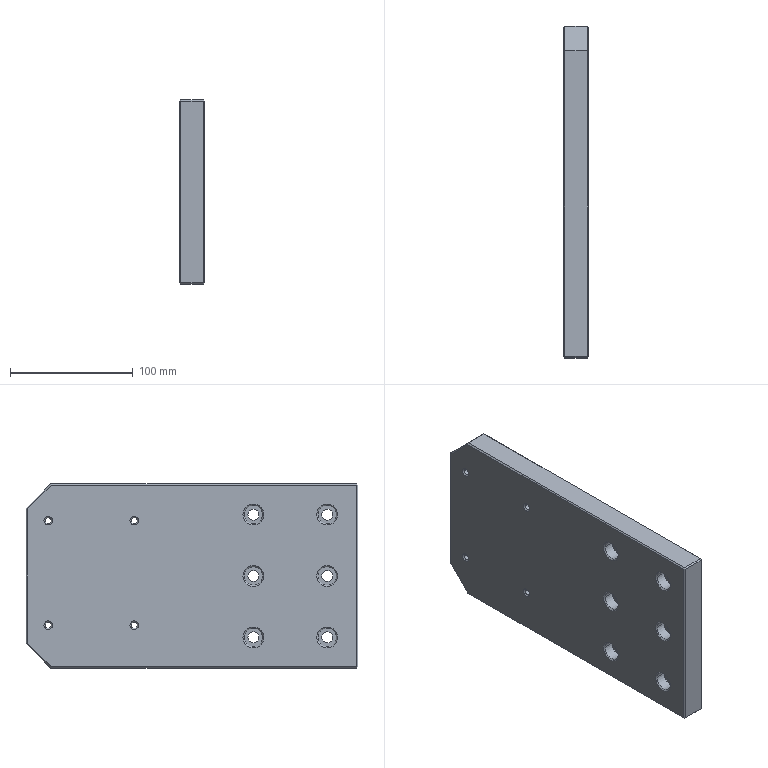Component | SolidWorks | CutterFixingPlateA-1 | 1 solid | 104 faces | box 20 x 270 x 150 mm | volume 785545 mm3 | cone 40 | cylinder 32 | plane 32 | commonest cylinder face diameters 15 x12 9 x12 5 x8 | material 1060 Alloy
build123d program:
from build123d import *

# Parameters (mm, degrees)
BOSS_EXTRUDE1_DEPTH                                = 20
M6_TAPPED_HOLE1_D                                  = 5
CHAMFER1_SIZE                                      = 20
SKETCH6_W                                          = 478.656
SKETCH6_H                                          = 357.372
CUT_EXTRUDE1_DEPTH                                 = 463.52
HOLE_SIZE_ACCORDING_TO_TYPE_OF_HEXAGON_D           = 9
HOLE_SIZE_ACCORDING_TO_TYPE_OF_HEXAGON_CBORE_D     = 15
HOLE_SIZE_ACCORDING_TO_TYPE_OF_HEXAGON_CBORE_DEPTH = 9
CHAMFER2_SIZE                                      = 1


with BuildPart() as part:
    # Sketch1 → Boss-Extrude1 (new body)
    with BuildSketch(Plane.XY):
        Polygon((0, 0), (0, 375), (270, 375), (270, 225), (100, 225), (100, 85), (270, 85), (270, -90), (110, -90), (110, 0), align=None)
    extrude(amount=BOSS_EXTRUDE1_DEPTH)

    # M6 Tapped Hole1 (through all)
    with Locations(Plane.XY.offset(20)):
        with Locations((182, 340), (252, 340), (252, 9), (182, 9), (182, 255), (252, 255), (252, -76), (182, -76)):
            Hole(M6_TAPPED_HOLE1_D / 2)

    # Chamfer1
    chamfer1_edges = [part.edges().sort_by_distance(p)[0] for p in [
        (270, 375, 10),
        (270, 225, 10),
        (100, 225, 10),
        (100, 85, 10),
        (270, 85, 10),
        (110, -90, 10),
    ]]
    chamfer(chamfer1_edges, length=CHAMFER1_SIZE)

    # Sketch6 → Cut-Extrude1 (cut, through all)
    with BuildSketch(Plane.XY.offset(20)):
        with Locations((150.639, 46.314)):
            Rectangle(SKETCH6_W, SKETCH6_H)
    extrude(amount=-CUT_EXTRUDE1_DEPTH, mode=Mode.SUBTRACT)

    # Hole Size _according to_ type of Hexagon (through all)
    with Locations(Plane.XY.offset(20)):
        with Locations((25, 350), (25, 300), (25, 250), (85, 350), (85, 300), (85, 250)):
            CounterBoreHole(HOLE_SIZE_ACCORDING_TO_TYPE_OF_HEXAGON_D / 2, HOLE_SIZE_ACCORDING_TO_TYPE_OF_HEXAGON_CBORE_D / 2, HOLE_SIZE_ACCORDING_TO_TYPE_OF_HEXAGON_CBORE_DEPTH)

    # Chamfer2
    chamfer2_edges = [part.edges().sort_by_distance(p)[0] for p in [
        (0, 225, 10),
        (77.5, 250, 20),
        (89.5, 250, 0),
        (0, 375, 10),
        (77.5, 300, 20),
        (89.5, 300, 0),
        (77.5, 350, 20),
        (89.5, 350, 0),
        (17.5, 250, 20),
        (29.5, 250, 0),
        (17.5, 300, 20),
        (29.5, 300, 0),
        (17.5, 350, 20),
        (29.5, 350, 0),
        (0, 300, 20),
        (254.5, 255, 20),
        (254.5, 255, 0),
        (184.5, 255, 20),
        (184.5, 255, 0),
        (254.5, 340, 20),
        (254.5, 340, 0),
        (184.5, 340, 20),
        (184.5, 340, 0),
        (125, 375, 0),
        (270, 300, 0),
        (125, 225, 0),
        (260, 235, 0),
        (260, 365, 0),
        (125, 225, 20),
        (270, 300, 20),
        (125, 375, 20),
        (260, 235, 20),
        (260, 365, 20),
        (0, 300, 0),
    ]]
    chamfer(chamfer2_edges, length=CHAMFER2_SIZE)


solid = part.part

# Placed as in the assembly
solid = solid.moved(Location((-144.666, 130.264, 197.5), (-90, -90, 0)))